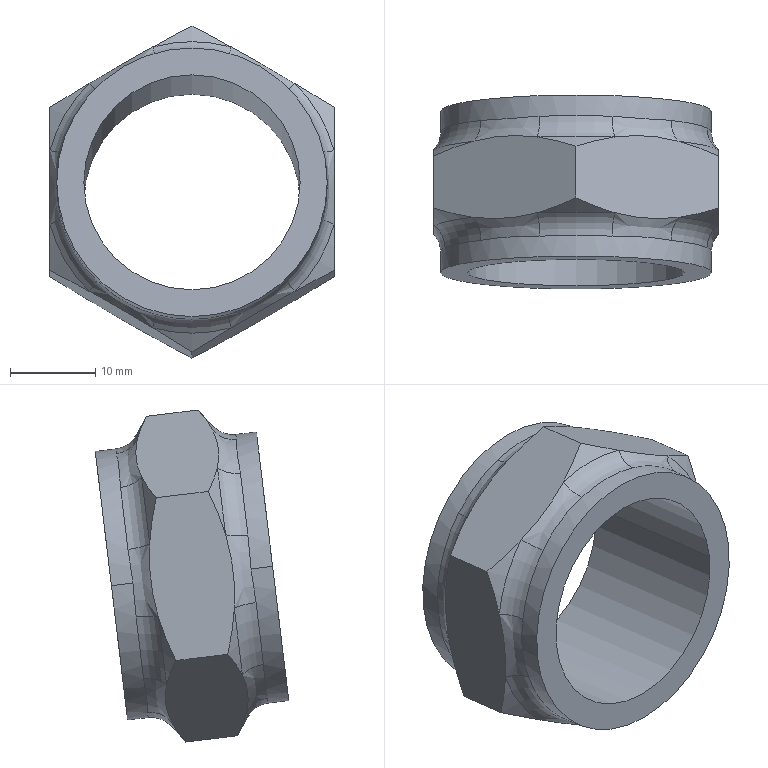Component | SolidWorks | DNR-71M20100BBEF2xx-A_504806-1_DNR-71M20100BBEF2xx-A_500791-1 | 1 solid | 50 faces | volume 7127 mm3 | cone 12 | spline 12 | torus 12 | plane 8 | cylinder 6 | commonest cylinder face diameters 31.75 x4 25.4 x2